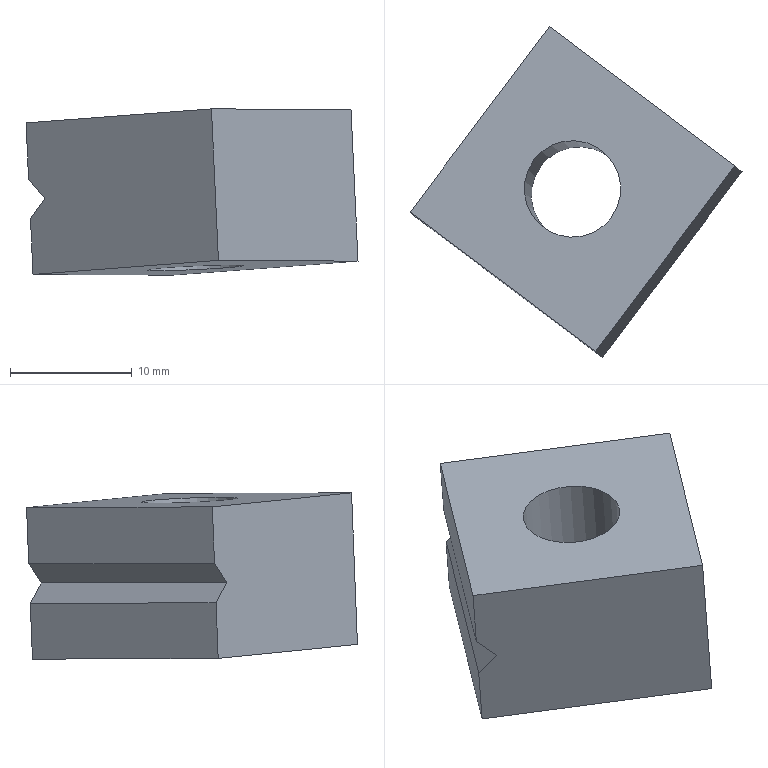Component | NX | MORDAZA_B | 1 solid | 10 faces | box 27.22 x 27.13 x 13.63 mm | volume 3854 mm3 | plane 9 | cylinder 1 | commonest cylinder face diameters 7.925 x1
STEP:
#1=CARTESIAN_POINT('',(0.,0.,0.));
#2=DIRECTION('',(0.,0.,1.));
#3=DIRECTION('',(1.,0.,0.));
#4=AXIS2_PLACEMENT_3D('',#1,#2,#3);
#5=CARTESIAN_POINT('',(19.853,1.252,2.373));
#6=VERTEX_POINT('',#5);
#7=CARTESIAN_POINT('',(8.411,-13.978,2.435));
#8=VERTEX_POINT('',#7);
#9=CARTESIAN_POINT('',(22.142,4.299,2.361));
#10=DIRECTION('',(-0.6006,-0.7995,0.003254));
#11=VECTOR('',#10,1.);
#12=LINE('',#9,#11);
#13=CARTESIAN_POINT('',(19.489,1.558,10.233));
#14=DIRECTION('',(0.7982,-0.5994,0.06028));
#15=DIRECTION('',(0.04625,-0.03881,-0.9982));
#16=AXIS2_PLACEMENT_3D('',#13,#14,#15);
#17=PLANE('',#16);
#18=CARTESIAN_POINT('',(7.874,3.81));
#19=DIRECTION('',(-0.,-1.));
#20=VECTOR('',#19,1.);
#21=LINE('',#18,#20);
#22=(GEOMETRIC_REPRESENTATION_CONTEXT(2)PARAMETRIC_REPRESENTATION_CONTEXT()REPRESENTATION_CONTEXT('',''));
#23=DEFINITIONAL_REPRESENTATION('',(#21),#22);
#24=PCURVE('',#17,#23);
#25=CARTESIAN_POINT('',(22.142,4.299,2.361));
#26=DIRECTION('',(0.5971,-0.4513,-0.6632));
#27=DIRECTION('',(-0.5317,0.3964,-0.7484));
#28=AXIS2_PLACEMENT_3D('',#25,#26,#27);
#29=PLANE('',#28);
#30=CARTESIAN_POINT('',(0.,0.));
#31=DIRECTION('',(0.,-1.));
#32=VECTOR('',#31,1.);
#33=LINE('',#30,#32);
#34=(GEOMETRIC_REPRESENTATION_CONTEXT(2)PARAMETRIC_REPRESENTATION_CONTEXT()REPRESENTATION_CONTEXT('',''));
#35=DEFINITIONAL_REPRESENTATION('',(#33),#34);
#36=PCURVE('',#29,#35);
#37=SURFACE_CURVE('',#12,(#24,#36),.PCURVE_S1.);
#38=EDGE_CURVE('',#6,#8,#37,.T.);
#39=ORIENTED_EDGE('',*,*,#38,.F.);
#40=CARTESIAN_POINT('',(20.065,1.075,-2.191));
#41=VERTEX_POINT('',#40);
#42=CARTESIAN_POINT('',(19.489,1.558,10.233));
#43=DIRECTION('',(0.04625,-0.03881,-0.9982));
#44=VECTOR('',#43,1.);
#45=LINE('',#42,#44);
#46=CARTESIAN_POINT('',(0.,0.));
#47=DIRECTION('',(1.,0.));
#48=VECTOR('',#47,1.);
#49=LINE('',#46,#48);
#50=(GEOMETRIC_REPRESENTATION_CONTEXT(2)PARAMETRIC_REPRESENTATION_CONTEXT()REPRESENTATION_CONTEXT('',''));
#51=DEFINITIONAL_REPRESENTATION('',(#49),#50);
#52=PCURVE('',#17,#51);
#53=CARTESIAN_POINT('',(34.694,-9.86,11.381));
#54=DIRECTION('',(-0.6006,-0.7995,0.003254));
#55=DIRECTION('',(0.04625,-0.03881,-0.9982));
#56=AXIS2_PLACEMENT_3D('',#53,#54,#55);
#57=PLANE('',#56);
#58=CARTESIAN_POINT('',(-0.,-19.05));
#59=DIRECTION('',(1.,0.));
#60=VECTOR('',#59,1.);
#61=LINE('',#58,#60);
#62=(GEOMETRIC_REPRESENTATION_CONTEXT(2)PARAMETRIC_REPRESENTATION_CONTEXT()REPRESENTATION_CONTEXT('',''));
#63=DEFINITIONAL_REPRESENTATION('',(#61),#62);
#64=PCURVE('',#57,#63);
#65=SURFACE_CURVE('',#45,(#52,#64),.PCURVE_S1.);
#66=EDGE_CURVE('',#6,#41,#65,.T.);
#67=ORIENTED_EDGE('',*,*,#66,.T.);
#68=CARTESIAN_POINT('',(8.622,-14.156,-2.129));
#69=VERTEX_POINT('',#68);
#70=CARTESIAN_POINT('',(20.065,1.075,-2.191));
#71=DIRECTION('',(-0.6006,-0.7995,0.003254));
#72=VECTOR('',#71,1.);
#73=LINE('',#70,#72);
#74=CARTESIAN_POINT('',(12.446,-0.));
#75=DIRECTION('',(-0.,-1.));
#76=VECTOR('',#75,1.);
#77=LINE('',#74,#76);
#78=(GEOMETRIC_REPRESENTATION_CONTEXT(2)PARAMETRIC_REPRESENTATION_CONTEXT()REPRESENTATION_CONTEXT('',''));
#79=DEFINITIONAL_REPRESENTATION('',(#77),#78);
#80=PCURVE('',#17,#79);
#81=CARTESIAN_POINT('',(8.622,-14.156,-2.129));
#82=DIRECTION('',(-0.04625,0.03881,0.9982));
#83=DIRECTION('',(0.7982,-0.5994,0.06028));
#84=AXIS2_PLACEMENT_3D('',#81,#82,#83);
#85=PLANE('',#84);
#86=CARTESIAN_POINT('',(-0.,19.05));
#87=DIRECTION('',(-0.,-1.));
#88=VECTOR('',#87,1.);
#89=LINE('',#86,#88);
#90=(GEOMETRIC_REPRESENTATION_CONTEXT(2)PARAMETRIC_REPRESENTATION_CONTEXT()REPRESENTATION_CONTEXT('',''));
#91=DEFINITIONAL_REPRESENTATION('',(#89),#90);
#92=PCURVE('',#85,#91);
#93=SURFACE_CURVE('',#73,(#80,#92),.PCURVE_S1.);
#94=EDGE_CURVE('',#41,#69,#93,.T.);
#95=ORIENTED_EDGE('',*,*,#94,.T.);
#96=CARTESIAN_POINT('',(8.047,-13.673,10.295));
#97=DIRECTION('',(0.04625,-0.03881,-0.9982));
#98=VECTOR('',#97,1.);
#99=LINE('',#96,#98);
#100=CARTESIAN_POINT('',(0.,-19.05));
#101=DIRECTION('',(1.,0.));
#102=VECTOR('',#101,1.);
#103=LINE('',#100,#102);
#104=(GEOMETRIC_REPRESENTATION_CONTEXT(2)PARAMETRIC_REPRESENTATION_CONTEXT()REPRESENTATION_CONTEXT('',''));
#105=DEFINITIONAL_REPRESENTATION('',(#103),#104);
#106=PCURVE('',#17,#105);
#107=CARTESIAN_POINT('',(8.047,-13.673,10.295));
#108=DIRECTION('',(0.6006,0.7995,-0.003254));
#109=DIRECTION('',(-0.04625,0.03881,0.9982));
#110=AXIS2_PLACEMENT_3D('',#107,#108,#109);
#111=PLANE('',#110);
#112=CARTESIAN_POINT('',(0.,0.));
#113=DIRECTION('',(-1.,0.));
#114=VECTOR('',#113,1.);
#115=LINE('',#112,#114);
#116=(GEOMETRIC_REPRESENTATION_CONTEXT(2)PARAMETRIC_REPRESENTATION_CONTEXT()REPRESENTATION_CONTEXT('',''));
#117=DEFINITIONAL_REPRESENTATION('',(#115),#116);
#118=PCURVE('',#111,#117);
#119=SURFACE_CURVE('',#99,(#106,#118),.PCURVE_S1.);
#120=EDGE_CURVE('',#8,#69,#119,.T.);
#121=ORIENTED_EDGE('',*,*,#120,.F.);
#122=EDGE_LOOP('',(#39,#67,#95,#121));
#123=FACE_BOUND('',#122,.T.);
#124=ADVANCED_FACE('',(#123),#17,.F.);
#125=CARTESIAN_POINT('',(9.605,-14.868,4.115));
#126=VERTEX_POINT('',#125);
#127=CARTESIAN_POINT('',(8.411,-13.978,2.435));
#128=DIRECTION('',(0.5317,-0.3964,0.7484));
#129=VECTOR('',#128,1.);
#130=LINE('',#127,#129);
#131=CARTESIAN_POINT('',(-7.874,-0.));
#132=DIRECTION('',(0.7071,0.7071));
#133=VECTOR('',#132,1.);
#134=LINE('',#131,#133);
#135=(GEOMETRIC_REPRESENTATION_CONTEXT(2)PARAMETRIC_REPRESENTATION_CONTEXT()REPRESENTATION_CONTEXT('',''));
#136=DEFINITIONAL_REPRESENTATION('',(#134),#135);
#137=PCURVE('',#111,#136);
#138=CARTESIAN_POINT('',(0.,-22.86));
#139=DIRECTION('',(-1.,0.));
#140=VECTOR('',#139,1.);
#141=LINE('',#138,#140);
#142=(GEOMETRIC_REPRESENTATION_CONTEXT(2)PARAMETRIC_REPRESENTATION_CONTEXT()REPRESENTATION_CONTEXT('',''));
#143=DEFINITIONAL_REPRESENTATION('',(#141),#142);
#144=PCURVE('',#29,#143);
#145=SURFACE_CURVE('',#130,(#137,#144),.PCURVE_S1.);
#146=EDGE_CURVE('',#8,#126,#145,.T.);
#147=ORIENTED_EDGE('',*,*,#146,.F.);
#148=ORIENTED_EDGE('',*,*,#120,.T.);
#149=CARTESIAN_POINT('',(23.828,-25.574,-0.9802));
#150=VERTEX_POINT('',#149);
#151=CARTESIAN_POINT('',(8.622,-14.156,-2.129));
#152=DIRECTION('',(0.7982,-0.5994,0.06028));
#153=VECTOR('',#152,1.);
#154=LINE('',#151,#153);
#155=CARTESIAN_POINT('',(-12.446,-0.));
#156=DIRECTION('',(0.,1.));
#157=VECTOR('',#156,1.);
#158=LINE('',#155,#157);
#159=(GEOMETRIC_REPRESENTATION_CONTEXT(2)PARAMETRIC_REPRESENTATION_CONTEXT()REPRESENTATION_CONTEXT('',''));
#160=DEFINITIONAL_REPRESENTATION('',(#158),#159);
#161=PCURVE('',#111,#160);
#162=CARTESIAN_POINT('',(0.,0.));
#163=DIRECTION('',(1.,0.));
#164=VECTOR('',#163,1.);
#165=LINE('',#162,#164);
#166=(GEOMETRIC_REPRESENTATION_CONTEXT(2)PARAMETRIC_REPRESENTATION_CONTEXT()REPRESENTATION_CONTEXT('',''));
#167=DEFINITIONAL_REPRESENTATION('',(#165),#166);
#168=PCURVE('',#85,#167);
#169=SURFACE_CURVE('',#154,(#161,#168),.PCURVE_S1.);
#170=EDGE_CURVE('',#69,#150,#169,.T.);
#171=ORIENTED_EDGE('',*,*,#170,.T.);
#172=CARTESIAN_POINT('',(23.252,-25.091,11.443));
#173=VERTEX_POINT('',#172);
#174=CARTESIAN_POINT('',(23.252,-25.091,11.443));
#175=DIRECTION('',(0.04625,-0.03881,-0.9982));
#176=VECTOR('',#175,1.);
#177=LINE('',#174,#176);
#178=CARTESIAN_POINT('',(0.,19.05));
#179=DIRECTION('',(-1.,0.));
#180=VECTOR('',#179,1.);
#181=LINE('',#178,#180);
#182=(GEOMETRIC_REPRESENTATION_CONTEXT(2)PARAMETRIC_REPRESENTATION_CONTEXT()REPRESENTATION_CONTEXT('',''));
#183=DEFINITIONAL_REPRESENTATION('',(#181),#182);
#184=PCURVE('',#111,#183);
#185=CARTESIAN_POINT('',(23.252,-25.091,11.443));
#186=DIRECTION('',(-0.7982,0.5994,-0.06028));
#187=DIRECTION('',(-0.04625,0.03881,0.9982));
#188=AXIS2_PLACEMENT_3D('',#185,#186,#187);
#189=PLANE('',#188);
#190=CARTESIAN_POINT('',(0.,0.));
#191=DIRECTION('',(-1.,0.));
#192=VECTOR('',#191,1.);
#193=LINE('',#190,#192);
#194=(GEOMETRIC_REPRESENTATION_CONTEXT(2)PARAMETRIC_REPRESENTATION_CONTEXT()REPRESENTATION_CONTEXT('',''));
#195=DEFINITIONAL_REPRESENTATION('',(#193),#194);
#196=PCURVE('',#189,#195);
#197=SURFACE_CURVE('',#177,(#184,#196),.PCURVE_S1.);
#198=EDGE_CURVE('',#173,#150,#197,.T.);
#199=ORIENTED_EDGE('',*,*,#198,.F.);
#200=CARTESIAN_POINT('',(8.047,-13.673,10.295));
#201=VERTEX_POINT('',#200);
#202=CARTESIAN_POINT('',(8.047,-13.673,10.295));
#203=DIRECTION('',(0.7982,-0.5994,0.06028));
#204=VECTOR('',#203,1.);
#205=LINE('',#202,#204);
#206=CARTESIAN_POINT('',(0.,0.));
#207=DIRECTION('',(0.,1.));
#208=VECTOR('',#207,1.);
#209=LINE('',#206,#208);
#210=(GEOMETRIC_REPRESENTATION_CONTEXT(2)PARAMETRIC_REPRESENTATION_CONTEXT()REPRESENTATION_CONTEXT('',''));
#211=DEFINITIONAL_REPRESENTATION('',(#209),#210);
#212=PCURVE('',#111,#211);
#213=CARTESIAN_POINT('',(8.047,-13.673,10.295));
#214=DIRECTION('',(-0.04625,0.03881,0.9982));
#215=DIRECTION('',(0.7982,-0.5994,0.06028));
#216=AXIS2_PLACEMENT_3D('',#213,#214,#215);
#217=PLANE('',#216);
#218=CARTESIAN_POINT('',(0.,0.));
#219=DIRECTION('',(1.,0.));
#220=VECTOR('',#219,1.);
#221=LINE('',#218,#220);
#222=(GEOMETRIC_REPRESENTATION_CONTEXT(2)PARAMETRIC_REPRESENTATION_CONTEXT()REPRESENTATION_CONTEXT('',''));
#223=DEFINITIONAL_REPRESENTATION('',(#221),#222);
#224=PCURVE('',#217,#223);
#225=SURFACE_CURVE('',#205,(#212,#224),.PCURVE_S1.);
#226=EDGE_CURVE('',#201,#173,#225,.T.);
#227=ORIENTED_EDGE('',*,*,#226,.F.);
#228=CARTESIAN_POINT('',(8.26,-13.852,5.686));
#229=VERTEX_POINT('',#228);
#230=CARTESIAN_POINT('',(8.047,-13.673,10.295));
#231=DIRECTION('',(0.04625,-0.03881,-0.9982));
#232=VECTOR('',#231,1.);
#233=LINE('',#230,#232);
#234=CARTESIAN_POINT('',(0.,0.));
#235=DIRECTION('',(-1.,0.));
#236=VECTOR('',#235,1.);
#237=LINE('',#234,#236);
#238=(GEOMETRIC_REPRESENTATION_CONTEXT(2)PARAMETRIC_REPRESENTATION_CONTEXT()REPRESENTATION_CONTEXT('',''));
#239=DEFINITIONAL_REPRESENTATION('',(#237),#238);
#240=PCURVE('',#111,#239);
#241=CARTESIAN_POINT('',(19.489,1.558,10.233));
#242=DIRECTION('',(0.7982,-0.5994,0.06028));
#243=DIRECTION('',(0.04625,-0.03881,-0.9982));
#244=AXIS2_PLACEMENT_3D('',#241,#242,#243);
#245=PLANE('',#244);
#246=CARTESIAN_POINT('',(0.,-19.05));
#247=DIRECTION('',(1.,0.));
#248=VECTOR('',#247,1.);
#249=LINE('',#246,#248);
#250=(GEOMETRIC_REPRESENTATION_CONTEXT(2)PARAMETRIC_REPRESENTATION_CONTEXT()REPRESENTATION_CONTEXT('',''));
#251=DEFINITIONAL_REPRESENTATION('',(#249),#250);
#252=PCURVE('',#245,#251);
#253=SURFACE_CURVE('',#233,(#240,#252),.PCURVE_S1.);
#254=EDGE_CURVE('',#201,#229,#253,.T.);
#255=ORIENTED_EDGE('',*,*,#254,.T.);
#256=CARTESIAN_POINT('',(9.605,-14.868,4.115));
#257=DIRECTION('',(-0.5836,0.4412,0.6817));
#258=VECTOR('',#257,1.);
#259=LINE('',#256,#258);
#260=CARTESIAN_POINT('',(-6.287,1.587));
#261=DIRECTION('',(0.7246,-0.6892));
#262=VECTOR('',#261,1.);
#263=LINE('',#260,#262);
#264=(GEOMETRIC_REPRESENTATION_CONTEXT(2)PARAMETRIC_REPRESENTATION_CONTEXT()REPRESENTATION_CONTEXT('',''));
#265=DEFINITIONAL_REPRESENTATION('',(#263),#264);
#266=PCURVE('',#111,#265);
#267=CARTESIAN_POINT('',(23.335,3.409,4.041));
#268=DIRECTION('',(0.5465,-0.4076,0.7316));
#269=DIRECTION('',(0.5836,-0.4412,-0.6817));
#270=AXIS2_PLACEMENT_3D('',#267,#268,#269);
#271=PLANE('',#270);
#272=CARTESIAN_POINT('',(-0.,-22.86));
#273=DIRECTION('',(-1.,0.));
#274=VECTOR('',#273,1.);
#275=LINE('',#272,#274);
#276=(GEOMETRIC_REPRESENTATION_CONTEXT(2)PARAMETRIC_REPRESENTATION_CONTEXT()REPRESENTATION_CONTEXT('',''));
#277=DEFINITIONAL_REPRESENTATION('',(#275),#276);
#278=PCURVE('',#271,#277);
#279=SURFACE_CURVE('',#259,(#266,#278),.PCURVE_S1.);
#280=EDGE_CURVE('',#126,#229,#279,.T.);
#281=ORIENTED_EDGE('',*,*,#280,.F.);
#282=EDGE_LOOP('',(#147,#148,#171,#199,#227,#255,#281));
#283=FACE_BOUND('',#282,.T.);
#284=ADVANCED_FACE('',(#283),#111,.F.);
#285=CARTESIAN_POINT('',(19.489,1.558,10.233));
#286=VERTEX_POINT('',#285);
#287=CARTESIAN_POINT('',(19.703,1.379,5.624));
#288=VERTEX_POINT('',#287);
#289=CARTESIAN_POINT('',(19.489,1.558,10.233));
#290=DIRECTION('',(0.04625,-0.03881,-0.9982));
#291=VECTOR('',#290,1.);
#292=LINE('',#289,#291);
#293=CARTESIAN_POINT('',(0.,0.));
#294=DIRECTION('',(1.,0.));
#295=VECTOR('',#294,1.);
#296=LINE('',#293,#295);
#297=(GEOMETRIC_REPRESENTATION_CONTEXT(2)PARAMETRIC_REPRESENTATION_CONTEXT()REPRESENTATION_CONTEXT('',''));
#298=DEFINITIONAL_REPRESENTATION('',(#296),#297);
#299=PCURVE('',#245,#298);
#300=CARTESIAN_POINT('',(-0.,-19.05));
#301=DIRECTION('',(1.,0.));
#302=VECTOR('',#301,1.);
#303=LINE('',#300,#302);
#304=(GEOMETRIC_REPRESENTATION_CONTEXT(2)PARAMETRIC_REPRESENTATION_CONTEXT()REPRESENTATION_CONTEXT('',''));
#305=DEFINITIONAL_REPRESENTATION('',(#303),#304);
#306=PCURVE('',#57,#305);
#307=SURFACE_CURVE('',#292,(#299,#306),.PCURVE_S1.);
#308=EDGE_CURVE('',#286,#288,#307,.T.);
#309=ORIENTED_EDGE('',*,*,#308,.T.);
#310=CARTESIAN_POINT('',(21.991,4.425,5.611));
#311=DIRECTION('',(-0.6006,-0.7995,0.003254));
#312=VECTOR('',#311,1.);
#313=LINE('',#310,#312);
#314=CARTESIAN_POINT('',(4.617,3.81));
#315=DIRECTION('',(-0.,-1.));
#316=VECTOR('',#315,1.);
#317=LINE('',#314,#316);
#318=(GEOMETRIC_REPRESENTATION_CONTEXT(2)PARAMETRIC_REPRESENTATION_CONTEXT()REPRESENTATION_CONTEXT('',''));
#319=DEFINITIONAL_REPRESENTATION('',(#317),#318);
#320=PCURVE('',#245,#319);
#321=CARTESIAN_POINT('',(-2.304,-0.));
#322=DIRECTION('',(0.,-1.));
#323=VECTOR('',#322,1.);
#324=LINE('',#321,#323);
#325=(GEOMETRIC_REPRESENTATION_CONTEXT(2)PARAMETRIC_REPRESENTATION_CONTEXT()REPRESENTATION_CONTEXT('',''));
#326=DEFINITIONAL_REPRESENTATION('',(#324),#325);
#327=PCURVE('',#271,#326);
#328=SURFACE_CURVE('',#313,(#320,#327),.PCURVE_S1.);
#329=EDGE_CURVE('',#288,#229,#328,.T.);
#330=ORIENTED_EDGE('',*,*,#329,.T.);
#331=ORIENTED_EDGE('',*,*,#254,.F.);
#332=CARTESIAN_POINT('',(19.489,1.558,10.233));
#333=DIRECTION('',(-0.6006,-0.7995,0.003254));
#334=VECTOR('',#333,1.);
#335=LINE('',#332,#334);
#336=CARTESIAN_POINT('',(0.,0.));
#337=DIRECTION('',(-0.,-1.));
#338=VECTOR('',#337,1.);
#339=LINE('',#336,#338);
#340=(GEOMETRIC_REPRESENTATION_CONTEXT(2)PARAMETRIC_REPRESENTATION_CONTEXT()REPRESENTATION_CONTEXT('',''));
#341=DEFINITIONAL_REPRESENTATION('',(#339),#340);
#342=PCURVE('',#245,#341);
#343=CARTESIAN_POINT('',(-0.,19.05));
#344=DIRECTION('',(-0.,-1.));
#345=VECTOR('',#344,1.);
#346=LINE('',#343,#345);
#347=(GEOMETRIC_REPRESENTATION_CONTEXT(2)PARAMETRIC_REPRESENTATION_CONTEXT()REPRESENTATION_CONTEXT('',''));
#348=DEFINITIONAL_REPRESENTATION('',(#346),#347);
#349=PCURVE('',#217,#348);
#350=SURFACE_CURVE('',#335,(#342,#349),.PCURVE_S1.);
#351=EDGE_CURVE('',#286,#201,#350,.T.);
#352=ORIENTED_EDGE('',*,*,#351,.F.);
#353=EDGE_LOOP('',(#309,#330,#331,#352));
#354=FACE_BOUND('',#353,.T.);
#355=ADVANCED_FACE('',(#354),#245,.F.);
#356=CARTESIAN_POINT('',(35.27,-10.343,-1.042));
#357=VERTEX_POINT('',#356);
#358=CARTESIAN_POINT('',(23.828,-25.574,-0.9802));
#359=DIRECTION('',(0.6006,0.7995,-0.003254));
#360=VECTOR('',#359,1.);
#361=LINE('',#358,#360);
#362=CARTESIAN_POINT('',(-12.446,0.));
#363=DIRECTION('',(-0.,1.));
#364=VECTOR('',#363,1.);
#365=LINE('',#362,#364);
#366=(GEOMETRIC_REPRESENTATION_CONTEXT(2)PARAMETRIC_REPRESENTATION_CONTEXT()REPRESENTATION_CONTEXT('',''));
#367=DEFINITIONAL_REPRESENTATION('',(#365),#366);
#368=PCURVE('',#189,#367);
#369=CARTESIAN_POINT('',(19.05,0.));
#370=DIRECTION('',(0.,1.));
#371=VECTOR('',#370,1.);
#372=LINE('',#369,#371);
#373=(GEOMETRIC_REPRESENTATION_CONTEXT(2)PARAMETRIC_REPRESENTATION_CONTEXT()REPRESENTATION_CONTEXT('',''));
#374=DEFINITIONAL_REPRESENTATION('',(#372),#373);
#375=PCURVE('',#85,#374);
#376=SURFACE_CURVE('',#361,(#368,#375),.PCURVE_S1.);
#377=EDGE_CURVE('',#150,#357,#376,.T.);
#378=ORIENTED_EDGE('',*,*,#377,.T.);
#379=CARTESIAN_POINT('',(34.694,-9.86,11.381));
#380=VERTEX_POINT('',#379);
#381=CARTESIAN_POINT('',(34.694,-9.86,11.381));
#382=DIRECTION('',(0.04625,-0.03881,-0.9982));
#383=VECTOR('',#382,1.);
#384=LINE('',#381,#383);
#385=CARTESIAN_POINT('',(-0.,19.05));
#386=DIRECTION('',(-1.,0.));
#387=VECTOR('',#386,1.);
#388=LINE('',#385,#387);
#389=(GEOMETRIC_REPRESENTATION_CONTEXT(2)PARAMETRIC_REPRESENTATION_CONTEXT()REPRESENTATION_CONTEXT('',''));
#390=DEFINITIONAL_REPRESENTATION('',(#388),#389);
#391=PCURVE('',#189,#390);
#392=CARTESIAN_POINT('',(0.,0.));
#393=DIRECTION('',(1.,0.));
#394=VECTOR('',#393,1.);
#395=LINE('',#392,#394);
#396=(GEOMETRIC_REPRESENTATION_CONTEXT(2)PARAMETRIC_REPRESENTATION_CONTEXT()REPRESENTATION_CONTEXT('',''));
#397=DEFINITIONAL_REPRESENTATION('',(#395),#396);
#398=PCURVE('',#57,#397);
#399=SURFACE_CURVE('',#384,(#391,#398),.PCURVE_S1.);
#400=EDGE_CURVE('',#380,#357,#399,.T.);
#401=ORIENTED_EDGE('',*,*,#400,.F.);
#402=CARTESIAN_POINT('',(23.252,-25.091,11.443));
#403=DIRECTION('',(0.6006,0.7995,-0.003254));
#404=VECTOR('',#403,1.);
#405=LINE('',#402,#404);
#406=CARTESIAN_POINT('',(0.,0.));
#407=DIRECTION('',(-0.,1.));
#408=VECTOR('',#407,1.);
#409=LINE('',#406,#408);
#410=(GEOMETRIC_REPRESENTATION_CONTEXT(2)PARAMETRIC_REPRESENTATION_CONTEXT()REPRESENTATION_CONTEXT('',''));
#411=DEFINITIONAL_REPRESENTATION('',(#409),#410);
#412=PCURVE('',#189,#411);
#413=CARTESIAN_POINT('',(19.05,-0.));
#414=DIRECTION('',(0.,1.));
#415=VECTOR('',#414,1.);
#416=LINE('',#413,#415);
#417=(GEOMETRIC_REPRESENTATION_CONTEXT(2)PARAMETRIC_REPRESENTATION_CONTEXT()REPRESENTATION_CONTEXT('',''));
#418=DEFINITIONAL_REPRESENTATION('',(#416),#417);
#419=PCURVE('',#217,#418);
#420=SURFACE_CURVE('',#405,(#412,#419),.PCURVE_S1.);
#421=EDGE_CURVE('',#173,#380,#420,.T.);
#422=ORIENTED_EDGE('',*,*,#421,.F.);
#423=ORIENTED_EDGE('',*,*,#198,.T.);
#424=EDGE_LOOP('',(#378,#401,#422,#423));
#425=FACE_BOUND('',#424,.T.);
#426=ADVANCED_FACE('',(#425),#189,.F.);
#427=ORIENTED_EDGE('',*,*,#66,.F.);
#428=CARTESIAN_POINT('',(21.047,0.3624,4.053));
#429=VERTEX_POINT('',#428);
#430=CARTESIAN_POINT('',(29.976,-6.294,16.622));
#431=DIRECTION('',(0.5317,-0.3964,0.7484));
#432=VECTOR('',#431,1.);
#433=LINE('',#430,#432);
#434=CARTESIAN_POINT('',(-5.588,-5.588));
#435=DIRECTION('',(-0.7071,0.7071));
#436=VECTOR('',#435,1.);
#437=LINE('',#434,#436);
#438=(GEOMETRIC_REPRESENTATION_CONTEXT(2)PARAMETRIC_REPRESENTATION_CONTEXT()REPRESENTATION_CONTEXT('',''));
#439=DEFINITIONAL_REPRESENTATION('',(#437),#438);
#440=PCURVE('',#57,#439);
#441=CARTESIAN_POINT('',(-19.038,-3.81));
#442=DIRECTION('',(-1.,0.));
#443=VECTOR('',#442,1.);
#444=LINE('',#441,#443);
#445=(GEOMETRIC_REPRESENTATION_CONTEXT(2)PARAMETRIC_REPRESENTATION_CONTEXT()REPRESENTATION_CONTEXT('',''));
#446=DEFINITIONAL_REPRESENTATION('',(#444),#445);
#447=PCURVE('',#29,#446);
#448=SURFACE_CURVE('',#433,(#440,#447),.PCURVE_S1.);
#449=EDGE_CURVE('',#6,#429,#448,.T.);
#450=ORIENTED_EDGE('',*,*,#449,.T.);
#451=CARTESIAN_POINT('',(25.412,-2.937,-1.046));
#452=DIRECTION('',(-0.5836,0.4412,0.6817));
#453=VECTOR('',#452,1.);
#454=LINE('',#451,#453);
#455=CARTESIAN_POINT('',(11.706,-12.308));
#456=DIRECTION('',(-0.7246,-0.6892));
#457=VECTOR('',#456,1.);
#458=LINE('',#455,#457);
#459=(GEOMETRIC_REPRESENTATION_CONTEXT(2)PARAMETRIC_REPRESENTATION_CONTEXT()REPRESENTATION_CONTEXT('',''));
#460=DEFINITIONAL_REPRESENTATION('',(#458),#459);
#461=PCURVE('',#57,#460);
#462=CARTESIAN_POINT('',(7.479,-3.81));
#463=DIRECTION('',(-1.,0.));
#464=VECTOR('',#463,1.);
#465=LINE('',#462,#464);
#466=(GEOMETRIC_REPRESENTATION_CONTEXT(2)PARAMETRIC_REPRESENTATION_CONTEXT()REPRESENTATION_CONTEXT('',''));
#467=DEFINITIONAL_REPRESENTATION('',(#465),#466);
#468=PCURVE('',#271,#467);
#469=SURFACE_CURVE('',#454,(#461,#468),.PCURVE_S1.);
#470=EDGE_CURVE('',#429,#288,#469,.T.);
#471=ORIENTED_EDGE('',*,*,#470,.T.);
#472=ORIENTED_EDGE('',*,*,#308,.F.);
#473=CARTESIAN_POINT('',(34.694,-9.86,11.381));
#474=DIRECTION('',(-0.7982,0.5994,-0.06028));
#475=VECTOR('',#474,1.);
#476=LINE('',#473,#475);
#477=CARTESIAN_POINT('',(0.,0.));
#478=DIRECTION('',(0.,-1.));
#479=VECTOR('',#478,1.);
#480=LINE('',#477,#479);
#481=(GEOMETRIC_REPRESENTATION_CONTEXT(2)PARAMETRIC_REPRESENTATION_CONTEXT()REPRESENTATION_CONTEXT('',''));
#482=DEFINITIONAL_REPRESENTATION('',(#480),#481);
#483=PCURVE('',#57,#482);
#484=CARTESIAN_POINT('',(19.05,19.05));
#485=DIRECTION('',(-1.,-0.));
#486=VECTOR('',#485,1.);
#487=LINE('',#484,#486);
#488=(GEOMETRIC_REPRESENTATION_CONTEXT(2)PARAMETRIC_REPRESENTATION_CONTEXT()REPRESENTATION_CONTEXT('',''));
#489=DEFINITIONAL_REPRESENTATION('',(#487),#488);
#490=PCURVE('',#217,#489);
#491=SURFACE_CURVE('',#476,(#483,#490),.PCURVE_S1.);
#492=EDGE_CURVE('',#380,#286,#491,.T.);
#493=ORIENTED_EDGE('',*,*,#492,.F.);
#494=ORIENTED_EDGE('',*,*,#400,.T.);
#495=CARTESIAN_POINT('',(35.27,-10.343,-1.042));
#496=DIRECTION('',(-0.7982,0.5994,-0.06028));
#497=VECTOR('',#496,1.);
#498=LINE('',#495,#497);
#499=CARTESIAN_POINT('',(12.446,0.));
#500=DIRECTION('',(0.,-1.));
#501=VECTOR('',#500,1.);
#502=LINE('',#499,#501);
#503=(GEOMETRIC_REPRESENTATION_CONTEXT(2)PARAMETRIC_REPRESENTATION_CONTEXT()REPRESENTATION_CONTEXT('',''));
#504=DEFINITIONAL_REPRESENTATION('',(#502),#503);
#505=PCURVE('',#57,#504);
#506=CARTESIAN_POINT('',(19.05,19.05));
#507=DIRECTION('',(-1.,-0.));
#508=VECTOR('',#507,1.);
#509=LINE('',#506,#508);
#510=(GEOMETRIC_REPRESENTATION_CONTEXT(2)PARAMETRIC_REPRESENTATION_CONTEXT()REPRESENTATION_CONTEXT('',''));
#511=DEFINITIONAL_REPRESENTATION('',(#509),#510);
#512=PCURVE('',#85,#511);
#513=SURFACE_CURVE('',#498,(#505,#512),.PCURVE_S1.);
#514=EDGE_CURVE('',#357,#41,#513,.T.);
#515=ORIENTED_EDGE('',*,*,#514,.T.);
#516=EDGE_LOOP('',(#427,#450,#471,#472,#493,#494,#515));
#517=FACE_BOUND('',#516,.T.);
#518=ADVANCED_FACE('',(#517),#57,.F.);
#519=CARTESIAN_POINT('',(24.533,-14.142,11.077));
#520=VERTEX_POINT('',#519);
#521=CARTESIAN_POINT('',(21.371,-11.767,10.838));
#522=DIRECTION('',(-0.04625,0.03881,0.9982));
#523=DIRECTION('',(0.7982,-0.5994,0.06028));
#524=AXIS2_PLACEMENT_3D('',#521,#522,#523);
#525=CIRCLE('',#524,3.962);
#526=CARTESIAN_POINT('',(9.525,9.525));
#527=DIRECTION('',(1.,-0.));
#528=AXIS2_PLACEMENT_2D('',#526,#527);
#529=CIRCLE('',#528,3.962);
#530=(GEOMETRIC_REPRESENTATION_CONTEXT(2)PARAMETRIC_REPRESENTATION_CONTEXT()REPRESENTATION_CONTEXT('',''));
#531=DEFINITIONAL_REPRESENTATION('',(#529),#530);
#532=PCURVE('',#217,#531);
#533=CARTESIAN_POINT('',(22.169,-12.437,-6.403));
#534=DIRECTION('',(-0.04625,0.03881,0.9982));
#535=DIRECTION('',(0.7982,-0.5994,0.06028));
#536=AXIS2_PLACEMENT_3D('',#533,#534,#535);
#537=CYLINDRICAL_SURFACE('',#536,3.962);
#538=CARTESIAN_POINT('',(0.,17.272));
#539=DIRECTION('',(1.,-0.));
#540=VECTOR('',#539,1.);
#541=LINE('',#538,#540);
#542=(GEOMETRIC_REPRESENTATION_CONTEXT(2)PARAMETRIC_REPRESENTATION_CONTEXT()REPRESENTATION_CONTEXT('',''));
#543=DEFINITIONAL_REPRESENTATION('',(#541),#542);
#544=PCURVE('',#537,#543);
#545=SURFACE_CURVE('',#525,(#532,#544),.PCURVE_S1.);
#546=EDGE_CURVE('',#520,#520,#545,.T.);
#547=ORIENTED_EDGE('',*,*,#546,.F.);
#548=EDGE_LOOP('',(#547));
#549=FACE_BOUND('',#548,.T.);
#550=ORIENTED_EDGE('',*,*,#351,.T.);
#551=ORIENTED_EDGE('',*,*,#226,.T.);
#552=ORIENTED_EDGE('',*,*,#421,.T.);
#553=ORIENTED_EDGE('',*,*,#492,.T.);
#554=EDGE_LOOP('',(#550,#551,#552,#553));
#555=FACE_BOUND('',#554,.T.);
#556=ADVANCED_FACE('',(#549,#555),#217,.T.);
#557=CARTESIAN_POINT('',(25.109,-14.625,-1.346));
#558=VERTEX_POINT('',#557);
#559=CARTESIAN_POINT('',(21.946,-12.25,-1.585));
#560=DIRECTION('',(-0.04625,0.03881,0.9982));
#561=DIRECTION('',(0.7982,-0.5994,0.06028));
#562=AXIS2_PLACEMENT_3D('',#559,#560,#561);
#563=CIRCLE('',#562,3.962);
#564=CARTESIAN_POINT('',(9.525,9.525));
#565=DIRECTION('',(1.,-0.));
#566=AXIS2_PLACEMENT_2D('',#564,#565);
#567=CIRCLE('',#566,3.962);
#568=(GEOMETRIC_REPRESENTATION_CONTEXT(2)PARAMETRIC_REPRESENTATION_CONTEXT()REPRESENTATION_CONTEXT('',''));
#569=DEFINITIONAL_REPRESENTATION('',(#567),#568);
#570=PCURVE('',#85,#569);
#571=CARTESIAN_POINT('',(0.,4.826));
#572=DIRECTION('',(1.,0.));
#573=VECTOR('',#572,1.);
#574=LINE('',#571,#573);
#575=(GEOMETRIC_REPRESENTATION_CONTEXT(2)PARAMETRIC_REPRESENTATION_CONTEXT()REPRESENTATION_CONTEXT('',''));
#576=DEFINITIONAL_REPRESENTATION('',(#574),#575);
#577=PCURVE('',#537,#576);
#578=SURFACE_CURVE('',#563,(#570,#577),.PCURVE_S1.);
#579=EDGE_CURVE('',#558,#558,#578,.T.);
#580=ORIENTED_EDGE('',*,*,#579,.T.);
#581=EDGE_LOOP('',(#580));
#582=FACE_BOUND('',#581,.T.);
#583=ORIENTED_EDGE('',*,*,#94,.F.);
#584=ORIENTED_EDGE('',*,*,#514,.F.);
#585=ORIENTED_EDGE('',*,*,#377,.F.);
#586=ORIENTED_EDGE('',*,*,#170,.F.);
#587=EDGE_LOOP('',(#583,#584,#585,#586));
#588=FACE_BOUND('',#587,.T.);
#589=ADVANCED_FACE('',(#582,#588),#85,.F.);
#590=ORIENTED_EDGE('',*,*,#546,.F.);
#591=CARTESIAN_POINT('',(25.109,-14.625,-1.346));
#592=CARTESIAN_POINT('',(24.533,-14.142,11.077));
#593=B_SPLINE_CURVE_WITH_KNOTS('',1,(#591,#592),.UNSPECIFIED.,.F.,.F.,(2,2),(4.826,17.272),.PIECEWISE_BEZIER_KNOTS.);
#594=CARTESIAN_POINT('',(0.,0.));
#595=DIRECTION('',(0.,1.));
#596=VECTOR('',#595,1.);
#597=LINE('',#594,#596);
#598=(GEOMETRIC_REPRESENTATION_CONTEXT(2)PARAMETRIC_REPRESENTATION_CONTEXT()REPRESENTATION_CONTEXT('',''));
#599=DEFINITIONAL_REPRESENTATION('',(#597),#598);
#600=PCURVE('',#537,#599);
#601=CARTESIAN_POINT('',(6.283,0.));
#602=DIRECTION('',(0.,1.));
#603=VECTOR('',#602,1.);
#604=LINE('',#601,#603);
#605=(GEOMETRIC_REPRESENTATION_CONTEXT(2)PARAMETRIC_REPRESENTATION_CONTEXT()REPRESENTATION_CONTEXT('',''));
#606=DEFINITIONAL_REPRESENTATION('',(#604),#605);
#607=PCURVE('',#537,#606);
#608=SEAM_CURVE('',#593,(#600,#607),.PCURVE_S1.);
#609=EDGE_CURVE('',#558,#520,#608,.T.);
#610=ORIENTED_EDGE('',*,*,#609,.F.);
#611=ORIENTED_EDGE('',*,*,#579,.T.);
#612=ORIENTED_EDGE('',*,*,#609,.T.);
#613=EDGE_LOOP('',(#590,#610,#611,#612));
#614=FACE_BOUND('',#613,.F.);
#615=ADVANCED_FACE('',(#614),#537,.F.);
#616=ORIENTED_EDGE('',*,*,#38,.T.);
#617=ORIENTED_EDGE('',*,*,#146,.T.);
#618=CARTESIAN_POINT('',(23.335,3.409,4.041));
#619=DIRECTION('',(0.6006,0.7995,-0.003254));
#620=VECTOR('',#619,1.);
#621=LINE('',#618,#620);
#622=CARTESIAN_POINT('',(-2.245,0.));
#623=DIRECTION('',(-0.,1.));
#624=VECTOR('',#623,1.);
#625=LINE('',#622,#624);
#626=(GEOMETRIC_REPRESENTATION_CONTEXT(2)PARAMETRIC_REPRESENTATION_CONTEXT()REPRESENTATION_CONTEXT('',''));
#627=DEFINITIONAL_REPRESENTATION('',(#625),#626);
#628=PCURVE('',#29,#627);
#629=CARTESIAN_POINT('',(0.,0.));
#630=DIRECTION('',(-0.,1.));
#631=VECTOR('',#630,1.);
#632=LINE('',#629,#631);
#633=(GEOMETRIC_REPRESENTATION_CONTEXT(2)PARAMETRIC_REPRESENTATION_CONTEXT()REPRESENTATION_CONTEXT('',''));
#634=DEFINITIONAL_REPRESENTATION('',(#632),#633);
#635=PCURVE('',#271,#634);
#636=SURFACE_CURVE('',#621,(#628,#635),.PCURVE_S1.);
#637=EDGE_CURVE('',#126,#429,#636,.T.);
#638=ORIENTED_EDGE('',*,*,#637,.T.);
#639=ORIENTED_EDGE('',*,*,#449,.F.);
#640=EDGE_LOOP('',(#616,#617,#638,#639));
#641=FACE_BOUND('',#640,.T.);
#642=ADVANCED_FACE('',(#641),#29,.F.);
#643=ORIENTED_EDGE('',*,*,#637,.F.);
#644=ORIENTED_EDGE('',*,*,#280,.T.);
#645=ORIENTED_EDGE('',*,*,#329,.F.);
#646=ORIENTED_EDGE('',*,*,#470,.F.);
#647=EDGE_LOOP('',(#643,#644,#645,#646));
#648=FACE_BOUND('',#647,.T.);
#649=ADVANCED_FACE('',(#648),#271,.F.);
#650=CLOSED_SHELL('',(#124,#284,#355,#426,#518,#556,#589,#615,#642,#649));
#651=MANIFOLD_SOLID_BREP('',#650);
#652=(LENGTH_UNIT()NAMED_UNIT(*)SI_UNIT(.MILLI.,.METRE.));
#653=UNCERTAINTY_MEASURE_WITH_UNIT(LENGTH_MEASURE(0.000001),#652,'','');
#654=(NAMED_UNIT(*)PLANE_ANGLE_UNIT()SI_UNIT($,.RADIAN.));
#655=(NAMED_UNIT(*)SI_UNIT($,.STERADIAN.)SOLID_ANGLE_UNIT());
#656=(GEOMETRIC_REPRESENTATION_CONTEXT(3)GLOBAL_UNCERTAINTY_ASSIGNED_CONTEXT((#653))GLOBAL_UNIT_ASSIGNED_CONTEXT((#652,#654,#655))REPRESENTATION_CONTEXT('',''));
#657=ADVANCED_BREP_SHAPE_REPRESENTATION('',(#4,#651),#656);